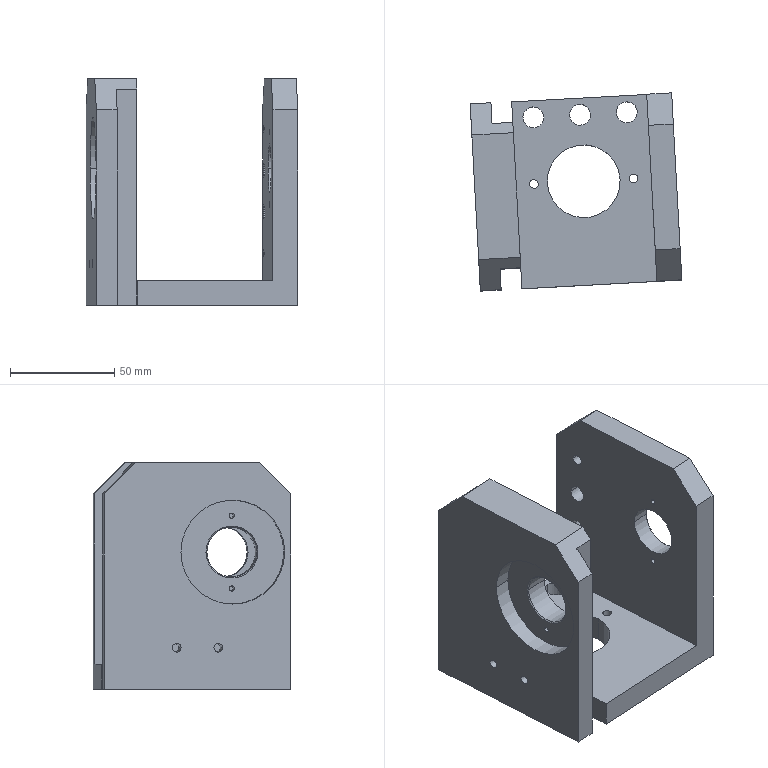Component | SolidWorks | BearingPressPartPLeft-1 | 1 solid | 68 faces | box 101.78 x 95.17 x 109 mm | volume 308409 mm3 | cylinder 40 | plane 24 | cone 4 | commonest cylinder face diameters 4.2 x8 2.5 x8 10 x6 8 x4 5 x4 50 x4 24 x4 35 x2
build123d program:
from build123d import *

# Parameters (mm, degrees)
BOSS_EXTRUDE1_DEPTH           = 90
SKETCH2_W                     = 133.192
SKETCH2_H                     = 10
CUT_EXTRUDE1_DEPTH            = 10
SKETCH3_W                     = 116.181
SKETCH3_H                     = 10
CUT_EXTRUDE2_DEPTH            = 10
CHAMFER1_2_SIZE               = 15
SKETCH5_R                     = 17.5
CUT_EXTRUDE4_DEPTH            = 165.067
SKETCH6_R                     = 12
CUT_EXTRUDE5_DEPTH            = 172.435
SKETCH7_R                     = 25
CUT_EXTRUDE6_DEPTH            = 3
CUT_EXTRUDE7_START            = -8.3
SKETCH8_R                     = 25
CUT_EXTRUDE7_DEPTH            = 8.3
M3_TAPPED_HOLE1_D             = 2.5
M10_TAPPED_HOLE1_D            = 10
M6_TAPPED_HOLE1_D             = 5
M6_TAPPED_HOLE1_DEPTH         = 15
M6_TAPPED_HOLE1_TIP           = 1.502
SIZE_MM_DOWEL_PIN_HOLE1_D     = 8
SIZE_MM_DOWEL_PIN_HOLE1_DEPTH = 15
SIZE_MM_DOWEL_PIN_HOLE1_TIP   = 2.403
M5_TAPPED_HOLE1_D             = 4.2
M5_TAPPED_HOLE1_DEPTH         = 20
M5_TAPPED_HOLE1_TIP           = 1.262
M5_TAPPED_HOLE2_D             = 4.2
CHAMFER1_SIZE                 = 0.5


with BuildPart() as part:
    # Sketch1 → Boss-Extrude1 (new body)
    with BuildSketch(Plane.XY):
        Polygon((109, 85), (12, 85), (12, 20), (109, 20), (109, 0), (0, 0), (0, 97), (109, 97), align=None)
    extrude(amount=BOSS_EXTRUDE1_DEPTH)

    # Sketch2 → Cut-Extrude1 (cut)
    with BuildSketch(Plane.XY.offset(90)):
        with Locations((42.404, 15)):
            Rectangle(SKETCH2_W, SKETCH2_H)
    extrude(amount=-CUT_EXTRUDE1_DEPTH, mode=Mode.SUBTRACT)

    # Sketch3 → Cut-Extrude2 (cut)
    with BuildSketch(Plane(origin=(0, 0, 0), x_dir=(-1, 0, 0), z_dir=(0, 0, -1))):
        with Locations((-50.91, 15)):
            Rectangle(SKETCH3_W, SKETCH3_H)
    extrude(amount=-CUT_EXTRUDE2_DEPTH, mode=Mode.SUBTRACT)

    # Chamfer1_2
    chamfer1_2_edges = [part.edges().sort_by_distance(p)[0] for p in [
        (109, 5, 0),
        (109, 91, 0),
        (109, 91, 90),
        (109, 5, 90),
    ]]
    chamfer(chamfer1_2_edges, length=CHAMFER1_2_SIZE)

    # Sketch5 → Cut-Extrude4 (cut, through all)
    with BuildSketch(Plane(origin=(12, 0, 0), x_dir=(0, 0, -1), z_dir=(1, 0, 0))):
        with Locations(Location((-50, 52.5, 0), (0, 0, 90))):
            Circle(SKETCH5_R)
    extrude(amount=-CUT_EXTRUDE4_DEPTH, mode=Mode.SUBTRACT)

    # Sketch6 → Cut-Extrude5 (cut, through all)
    with BuildSketch(Plane(origin=(0, 97, 0), x_dir=(1, 0, 0), z_dir=(0, 1, 0))):
        with Locations(Location((66, -28, 0), (0, 0, 270))):
            Circle(SKETCH6_R)
    extrude(amount=-CUT_EXTRUDE5_DEPTH, mode=Mode.SUBTRACT)

    # Sketch7 → Cut-Extrude6 (cut)
    with BuildSketch(Plane(origin=(0, 97, 0), x_dir=(1, 0, 0), z_dir=(0, 1, 0))):
        with Locations(Location((66, -28, 0), (0, 0, 270))):
            Circle(SKETCH7_R)
    extrude(amount=-CUT_EXTRUDE6_DEPTH, mode=Mode.SUBTRACT)

    # Sketch8 → Cut-Extrude7 (cut)
    with BuildSketch(Plane.XZ.offset(CUT_EXTRUDE7_START)):
        with Locations(Location((66, 28, 0), (0, 0, 90))):
            Circle(SKETCH8_R)
    extrude(amount=CUT_EXTRUDE7_DEPTH, mode=Mode.SUBTRACT)

    # M3 Tapped Hole1 (through all)
    with Locations(Plane(origin=(0, 94, 0), x_dir=(1, 0, 0), z_dir=(0, 1, 0))):
        with Locations((48.5, -28), (83.5, -28)):
            Hole(M3_TAPPED_HOLE1_D / 2)

    # M10 Tapped Hole1 (through all)
    with Locations(Plane(origin=(12, 0, 0), x_dir=(0, 0, -1), z_dir=(1, 0, 0))):
        with Locations((-82, 52.5), (-82, 30), (-82, 75)):
            Hole(M10_TAPPED_HOLE1_D / 2)

    # M6 Tapped Hole1
    with Locations(Plane(origin=(0, 97, 0), x_dir=(1, 0, 0), z_dir=(0, 1, 0))):
        with Locations((85, -76.87), (25, -76.87)):
            Hole(M6_TAPPED_HOLE1_D / 2, depth=M6_TAPPED_HOLE1_DEPTH)
            with Locations((0, 0, -(M6_TAPPED_HOLE1_DEPTH + M6_TAPPED_HOLE1_TIP / 2))):  # 118° drill point
                Cone(0, M6_TAPPED_HOLE1_D / 2, M6_TAPPED_HOLE1_TIP, mode=Mode.SUBTRACT)

    # Size mm Dowel Pin Hole1
    with Locations(Plane(origin=(0, 97, 0), x_dir=(1, 0, 0), z_dir=(0, 1, 0))):
        with Locations((65, -76.87), (45, -76.87)):
            Hole(SIZE_MM_DOWEL_PIN_HOLE1_D / 2, depth=SIZE_MM_DOWEL_PIN_HOLE1_DEPTH)
            with Locations((0, 0, -(SIZE_MM_DOWEL_PIN_HOLE1_DEPTH + SIZE_MM_DOWEL_PIN_HOLE1_TIP / 2))):  # 118° drill point
                Cone(0, SIZE_MM_DOWEL_PIN_HOLE1_D / 2, SIZE_MM_DOWEL_PIN_HOLE1_TIP, mode=Mode.SUBTRACT)

    # M5 Tapped Hole1
    with Locations(Plane(origin=(0, 0, 0), x_dir=(-1, 0, 0), z_dir=(0, -1, 0))):
        with Locations((-20, -55), (-20, -35)):
            Hole(M5_TAPPED_HOLE1_D / 2, depth=M5_TAPPED_HOLE1_DEPTH)
            with Locations((0, 0, -(M5_TAPPED_HOLE1_DEPTH + M5_TAPPED_HOLE1_TIP / 2))):  # 118° drill point
                Cone(0, M5_TAPPED_HOLE1_D / 2, M5_TAPPED_HOLE1_TIP, mode=Mode.SUBTRACT)

    # M5 Tapped Hole2 (through all)
    with Locations(Plane.ZY):
        with Locations((50, 76.5), (50, 28.5)):
            Hole(M5_TAPPED_HOLE2_D / 2)

    # Chamfer1
    chamfer1_edges = [part.edges().sort_by_distance(p)[0] for p in [
        (66, 94, 16),
        (66, 8.3, 16),
    ]]
    chamfer(chamfer1_edges, length=CHAMFER1_SIZE)


solid = part.part

# Placed as in the assembly
solid = solid.moved(Location((397.991, 75.166, -283.818), (-90, -3.137, -90)))